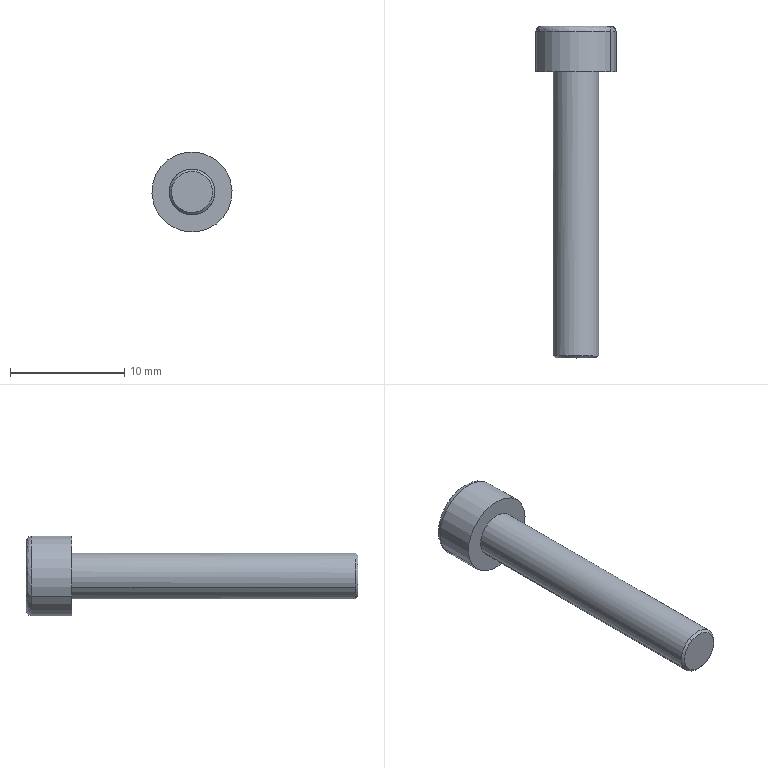Component | SolidWorks | M4X25-2 | 1 solid | 25 faces | box 7 x 29 x 7 mm | volume 449 mm3 | plane 15 | cylinder 4 | cone 4 | spline 2 | commonest cylinder face diameters 4 x2 7 x2 | material Standard Part
STEP:
#1=CARTESIAN_POINT('',(-0.3669,2.121,-0.7185));
#2=VERTEX_POINT('',#1);
#3=CARTESIAN_POINT('',(-0.6056,2.121,-0.8563));
#4=VERTEX_POINT('',#3);
#5=CARTESIAN_POINT('',(-0.4863,2.121,-0.7874));
#6=DIRECTION('',(-0.,-1.,0.));
#7=DIRECTION('',(0.866,0.,0.5));
#8=AXIS2_PLACEMENT_3D('',#5,#6,#7);
#9=CIRCLE('',#8,0.1378);
#10=EDGE_CURVE('',#2,#4,#9,.T.);
#11=ORIENTED_EDGE('',*,*,#10,.F.);
#12=CARTESIAN_POINT('',(-0.384,2.14,-0.7283));
#13=VERTEX_POINT('',#12);
#14=CARTESIAN_POINT('',(-0.384,2.121,-0.7283));
#15=DIRECTION('',(-0.5,0.,0.866));
#16=DIRECTION('',(0.866,0.,0.5));
#17=AXIS2_PLACEMENT_3D('',#14,#15,#16);
#18=CIRCLE('',#17,0.01969);
#19=EDGE_CURVE('',#2,#13,#18,.T.);
#20=ORIENTED_EDGE('',*,*,#19,.T.);
#21=CARTESIAN_POINT('',(-0.5885,2.14,-0.8465));
#22=VERTEX_POINT('',#21);
#23=CARTESIAN_POINT('',(-0.384,2.14,-0.7283));
#24=CARTESIAN_POINT('',(-0.5021,2.14,-0.5238));
#25=CARTESIAN_POINT('',(-0.7066,2.14,-0.6419));
#26=CARTESIAN_POINT('',(-0.5885,2.14,-0.8465));
#27=(BOUNDED_CURVE()B_SPLINE_CURVE(3,(#23,#24,#25,#26),.UNSPECIFIED.,.F.,.F.)B_SPLINE_CURVE_WITH_KNOTS((4,4),(0.,1.),.UNSPECIFIED.)CURVE()GEOMETRIC_REPRESENTATION_ITEM()RATIONAL_B_SPLINE_CURVE((1.,0.3333,0.3333,1.))REPRESENTATION_ITEM(''));
#28=EDGE_CURVE('',#13,#22,#27,.T.);
#29=ORIENTED_EDGE('',*,*,#28,.T.);
#30=CARTESIAN_POINT('',(-0.5885,2.121,-0.8465));
#31=DIRECTION('',(0.5,-0.,-0.866));
#32=DIRECTION('',(-0.866,0.,-0.5));
#33=AXIS2_PLACEMENT_3D('',#30,#31,#32);
#34=CIRCLE('',#33,0.01969);
#35=EDGE_CURVE('',#4,#22,#34,.T.);
#36=ORIENTED_EDGE('',*,*,#35,.F.);
#37=EDGE_LOOP('',(#11,#20,#29,#36));
#38=FACE_OUTER_BOUND('',#37,.T.);
#39=CARTESIAN_POINT('',(-0.3669,2.121,-0.7185));
#40=CARTESIAN_POINT('',(-0.5047,2.121,-0.4798));
#41=CARTESIAN_POINT('',(-0.7434,2.121,-0.6176));
#42=CARTESIAN_POINT('',(-0.6056,2.121,-0.8563));
#43=CARTESIAN_POINT('',(-0.3669,2.132,-0.7185));
#44=CARTESIAN_POINT('',(-0.5047,2.132,-0.4798));
#45=CARTESIAN_POINT('',(-0.7434,2.132,-0.6176));
#46=CARTESIAN_POINT('',(-0.6056,2.132,-0.8563));
#47=CARTESIAN_POINT('',(-0.374,2.14,-0.7226));
#48=CARTESIAN_POINT('',(-0.5036,2.14,-0.498));
#49=CARTESIAN_POINT('',(-0.7282,2.14,-0.6277));
#50=CARTESIAN_POINT('',(-0.5985,2.14,-0.8522));
#51=CARTESIAN_POINT('',(-0.384,2.14,-0.7283));
#52=CARTESIAN_POINT('',(-0.5021,2.14,-0.5238));
#53=CARTESIAN_POINT('',(-0.7066,2.14,-0.6419));
#54=CARTESIAN_POINT('',(-0.5885,2.14,-0.8465));
#55=(BOUNDED_SURFACE()B_SPLINE_SURFACE(3,3,((#39,#40,#41,#42),(#43,#44,#45,#46),(#47,#48,#49,#50),(#51,#52,#53,#54)),.UNSPECIFIED.,.F.,.F.,.T.)B_SPLINE_SURFACE_WITH_KNOTS((4,4),(4,4),(0.,1.),(0.,1.),.UNSPECIFIED.)GEOMETRIC_REPRESENTATION_ITEM()RATIONAL_B_SPLINE_SURFACE(((1.,0.3333,0.3333,1.),(0.8047,0.2682,0.2682,0.8047),(0.8047,0.2682,0.2682,0.8047),(1.,0.3333,0.3333,1.)))REPRESENTATION_ITEM('')SURFACE());
#56=ADVANCED_FACE('',(#38),#55,.T.);
#57=CARTESIAN_POINT('',(-0.4469,1.006,-0.8556));
#58=VERTEX_POINT('',#57);
#59=CARTESIAN_POINT('',(-0.5544,1.006,-0.8268));
#60=VERTEX_POINT('',#59);
#61=CARTESIAN_POINT('',(-0.4863,1.006,-0.7874));
#62=DIRECTION('',(0.,1.,-0.));
#63=DIRECTION('',(0.866,0.,0.5));
#64=AXIS2_PLACEMENT_3D('',#61,#62,#63);
#65=CIRCLE('',#64,0.07874);
#66=EDGE_CURVE('',#58,#60,#65,.T.);
#67=ORIENTED_EDGE('',*,*,#66,.T.);
#68=CARTESIAN_POINT('',(-0.5544,1.983,-0.8268));
#69=VERTEX_POINT('',#68);
#70=CARTESIAN_POINT('',(-0.5544,0.9986,-0.8268));
#71=DIRECTION('',(0.,1.,-0.));
#72=VECTOR('',#71,39.37);
#73=LINE('',#70,#72);
#74=EDGE_CURVE('',#60,#69,#73,.T.);
#75=ORIENTED_EDGE('',*,*,#74,.T.);
#76=CARTESIAN_POINT('',(-0.4181,1.983,-0.748));
#77=VERTEX_POINT('',#76);
#78=CARTESIAN_POINT('',(-0.4863,1.983,-0.7874));
#79=DIRECTION('',(-0.,-1.,0.));
#80=DIRECTION('',(0.866,0.,0.5));
#81=AXIS2_PLACEMENT_3D('',#78,#79,#80);
#82=CIRCLE('',#81,0.07874);
#83=EDGE_CURVE('',#69,#77,#82,.T.);
#84=ORIENTED_EDGE('',*,*,#83,.T.);
#85=CARTESIAN_POINT('',(-0.4181,1.006,-0.748));
#86=VERTEX_POINT('',#85);
#87=CARTESIAN_POINT('',(-0.4181,0.9986,-0.748));
#88=DIRECTION('',(0.,1.,-0.));
#89=VECTOR('',#88,39.37);
#90=LINE('',#87,#89);
#91=EDGE_CURVE('',#86,#77,#90,.T.);
#92=ORIENTED_EDGE('',*,*,#91,.F.);
#93=CARTESIAN_POINT('',(-0.4863,1.006,-0.7874));
#94=DIRECTION('',(0.,1.,-0.));
#95=DIRECTION('',(0.866,0.,0.5));
#96=AXIS2_PLACEMENT_3D('',#93,#94,#95);
#97=CIRCLE('',#96,0.07874);
#98=EDGE_CURVE('',#86,#58,#97,.T.);
#99=ORIENTED_EDGE('',*,*,#98,.T.);
#100=EDGE_LOOP('',(#67,#75,#84,#92,#99));
#101=FACE_OUTER_BOUND('',#100,.T.);
#102=CARTESIAN_POINT('',(-0.4863,0.9986,-0.7874));
#103=DIRECTION('',(0.,1.,-0.));
#104=DIRECTION('',(0.866,0.,0.5));
#105=AXIS2_PLACEMENT_3D('',#102,#103,#104);
#106=CYLINDRICAL_SURFACE('',#105,0.07874);
#107=ADVANCED_FACE('',(#101),#106,.T.);
#108=CARTESIAN_POINT('',(-0.5217,0.9986,-0.726));
#109=VERTEX_POINT('',#108);
#110=CARTESIAN_POINT('',(-0.4508,0.9986,-0.8488));
#111=VERTEX_POINT('',#110);
#112=CARTESIAN_POINT('',(-0.4863,0.9986,-0.7874));
#113=DIRECTION('',(-0.,1.,0.));
#114=DIRECTION('',(-0.5,0.,0.866));
#115=AXIS2_PLACEMENT_3D('',#112,#113,#114);
#116=CIRCLE('',#115,0.07087);
#117=EDGE_CURVE('',#109,#111,#116,.T.);
#118=ORIENTED_EDGE('',*,*,#117,.T.);
#119=CARTESIAN_POINT('',(-0.4469,1.006,-0.8556));
#120=DIRECTION('',(0.3536,0.7071,-0.6124));
#121=VECTOR('',#120,39.37);
#122=LINE('',#119,#121);
#123=EDGE_CURVE('',#111,#58,#122,.T.);
#124=ORIENTED_EDGE('',*,*,#123,.T.);
#125=ORIENTED_EDGE('',*,*,#98,.F.);
#126=CARTESIAN_POINT('',(-0.5256,1.006,-0.7192));
#127=VERTEX_POINT('',#126);
#128=CARTESIAN_POINT('',(-0.4863,1.006,-0.7874));
#129=DIRECTION('',(0.,1.,-0.));
#130=DIRECTION('',(0.866,0.,0.5));
#131=AXIS2_PLACEMENT_3D('',#128,#129,#130);
#132=CIRCLE('',#131,0.07874);
#133=EDGE_CURVE('',#127,#86,#132,.T.);
#134=ORIENTED_EDGE('',*,*,#133,.F.);
#135=CARTESIAN_POINT('',(-0.5256,1.006,-0.7192));
#136=DIRECTION('',(-0.3536,0.7071,0.6124));
#137=VECTOR('',#136,39.37);
#138=LINE('',#135,#137);
#139=EDGE_CURVE('',#109,#127,#138,.T.);
#140=ORIENTED_EDGE('',*,*,#139,.F.);
#141=EDGE_LOOP('',(#118,#124,#125,#134,#140));
#142=FACE_OUTER_BOUND('',#141,.T.);
#143=CARTESIAN_POINT('',(-0.4863,1.006,-0.7874));
#144=DIRECTION('',(-0.,1.,0.));
#145=DIRECTION('',(-0.5,0.,0.866));
#146=AXIS2_PLACEMENT_3D('',#143,#144,#145);
#147=CONICAL_SURFACE('',#146,0.07874,0.7854);
#148=ADVANCED_FACE('',(#142),#147,.T.);
#149=CARTESIAN_POINT('',(-0.6056,1.983,-0.8563));
#150=VERTEX_POINT('',#149);
#151=CARTESIAN_POINT('',(-0.3669,1.983,-0.7185));
#152=VERTEX_POINT('',#151);
#153=CARTESIAN_POINT('',(-0.4863,1.983,-0.7874));
#154=DIRECTION('',(-0.,-1.,0.));
#155=DIRECTION('',(0.866,0.,0.5));
#156=AXIS2_PLACEMENT_3D('',#153,#154,#155);
#157=CIRCLE('',#156,0.1378);
#158=EDGE_CURVE('',#150,#152,#157,.T.);
#159=ORIENTED_EDGE('',*,*,#158,.F.);
#160=CARTESIAN_POINT('',(-0.6056,1.983,-0.8563));
#161=DIRECTION('',(0.,1.,-0.));
#162=VECTOR('',#161,39.37);
#163=LINE('',#160,#162);
#164=EDGE_CURVE('',#150,#4,#163,.T.);
#165=ORIENTED_EDGE('',*,*,#164,.T.);
#166=CARTESIAN_POINT('',(-0.4863,2.121,-0.7874));
#167=DIRECTION('',(-0.,-1.,0.));
#168=DIRECTION('',(0.866,0.,0.5));
#169=AXIS2_PLACEMENT_3D('',#166,#167,#168);
#170=CIRCLE('',#169,0.1378);
#171=EDGE_CURVE('',#4,#2,#170,.T.);
#172=ORIENTED_EDGE('',*,*,#171,.T.);
#173=CARTESIAN_POINT('',(-0.3669,1.983,-0.7185));
#174=DIRECTION('',(0.,1.,-0.));
#175=VECTOR('',#174,39.37);
#176=LINE('',#173,#175);
#177=EDGE_CURVE('',#152,#2,#176,.T.);
#178=ORIENTED_EDGE('',*,*,#177,.F.);
#179=EDGE_LOOP('',(#159,#165,#172,#178));
#180=FACE_OUTER_BOUND('',#179,.T.);
#181=CARTESIAN_POINT('',(-0.4863,1.983,-0.7874));
#182=DIRECTION('',(0.,1.,-0.));
#183=DIRECTION('',(0.866,0.,0.5));
#184=AXIS2_PLACEMENT_3D('',#181,#182,#183);
#185=CYLINDRICAL_SURFACE('',#184,0.1378);
#186=ADVANCED_FACE('',(#180),#185,.T.);
#187=CARTESIAN_POINT('',(-0.4863,2.027,-0.7874));
#188=VERTEX_POINT('',#187);
#189=CARTESIAN_POINT('',(-0.4351,2.062,-0.7579));
#190=VERTEX_POINT('',#189);
#191=CARTESIAN_POINT('',(-0.4351,2.062,-0.7579));
#192=DIRECTION('',(0.75,0.5,0.433));
#193=VECTOR('',#192,39.37);
#194=LINE('',#191,#193);
#195=EDGE_CURVE('',#188,#190,#194,.T.);
#196=ORIENTED_EDGE('',*,*,#195,.F.);
#197=CARTESIAN_POINT('',(-0.5374,2.062,-0.8169));
#198=VERTEX_POINT('',#197);
#199=CARTESIAN_POINT('',(-0.5374,2.062,-0.8169));
#200=DIRECTION('',(-0.75,0.5,-0.433));
#201=VECTOR('',#200,39.37);
#202=LINE('',#199,#201);
#203=EDGE_CURVE('',#188,#198,#202,.T.);
#204=ORIENTED_EDGE('',*,*,#203,.T.);
#205=CARTESIAN_POINT('',(-0.5453,2.062,-0.7874));
#206=VERTEX_POINT('',#205);
#207=CARTESIAN_POINT('',(-0.4863,2.062,-0.7874));
#208=DIRECTION('',(-0.,-1.,0.));
#209=DIRECTION('',(0.866,0.,0.5));
#210=AXIS2_PLACEMENT_3D('',#207,#208,#209);
#211=CIRCLE('',#210,0.05906);
#212=EDGE_CURVE('',#206,#198,#211,.T.);
#213=ORIENTED_EDGE('',*,*,#212,.F.);
#214=CARTESIAN_POINT('',(-0.5158,2.062,-0.7363));
#215=VERTEX_POINT('',#214);
#216=CARTESIAN_POINT('',(-0.4863,2.062,-0.7874));
#217=DIRECTION('',(0.,1.,-0.));
#218=DIRECTION('',(0.866,0.,0.5));
#219=AXIS2_PLACEMENT_3D('',#216,#217,#218);
#220=CIRCLE('',#219,0.05906);
#221=EDGE_CURVE('',#206,#215,#220,.T.);
#222=ORIENTED_EDGE('',*,*,#221,.T.);
#223=CARTESIAN_POINT('',(-0.4567,2.062,-0.7363));
#224=VERTEX_POINT('',#223);
#225=CARTESIAN_POINT('',(-0.4863,2.062,-0.7874));
#226=DIRECTION('',(-0.,-1.,0.));
#227=DIRECTION('',(0.866,0.,0.5));
#228=AXIS2_PLACEMENT_3D('',#225,#226,#227);
#229=CIRCLE('',#228,0.05906);
#230=EDGE_CURVE('',#224,#215,#229,.T.);
#231=ORIENTED_EDGE('',*,*,#230,.F.);
#232=CARTESIAN_POINT('',(-0.4863,2.062,-0.7874));
#233=DIRECTION('',(-0.,-1.,0.));
#234=DIRECTION('',(0.866,0.,0.5));
#235=AXIS2_PLACEMENT_3D('',#232,#233,#234);
#236=CIRCLE('',#235,0.05906);
#237=EDGE_CURVE('',#190,#224,#236,.T.);
#238=ORIENTED_EDGE('',*,*,#237,.F.);
#239=EDGE_LOOP('',(#196,#204,#213,#222,#231,#238));
#240=FACE_OUTER_BOUND('',#239,.T.);
#241=CARTESIAN_POINT('',(-0.4863,2.062,-0.7874));
#242=DIRECTION('',(0.,1.,-0.));
#243=DIRECTION('',(0.866,0.,0.5));
#244=AXIS2_PLACEMENT_3D('',#241,#242,#243);
#245=CONICAL_SURFACE('',#244,0.05906,1.047);
#246=ADVANCED_FACE('',(#240),#245,.F.);
#247=ORIENTED_EDGE('',*,*,#74,.F.);
#248=CARTESIAN_POINT('',(-0.4863,1.006,-0.7874));
#249=DIRECTION('',(0.,1.,-0.));
#250=DIRECTION('',(0.866,0.,0.5));
#251=AXIS2_PLACEMENT_3D('',#248,#249,#250);
#252=CIRCLE('',#251,0.07874);
#253=EDGE_CURVE('',#60,#127,#252,.T.);
#254=ORIENTED_EDGE('',*,*,#253,.T.);
#255=ORIENTED_EDGE('',*,*,#133,.T.);
#256=ORIENTED_EDGE('',*,*,#91,.T.);
#257=CARTESIAN_POINT('',(-0.4863,1.983,-0.7874));
#258=DIRECTION('',(-0.,-1.,0.));
#259=DIRECTION('',(0.866,0.,0.5));
#260=AXIS2_PLACEMENT_3D('',#257,#258,#259);
#261=CIRCLE('',#260,0.07874);
#262=EDGE_CURVE('',#77,#69,#261,.T.);
#263=ORIENTED_EDGE('',*,*,#262,.T.);
#264=EDGE_LOOP('',(#247,#254,#255,#256,#263));
#265=FACE_OUTER_BOUND('',#264,.T.);
#266=CARTESIAN_POINT('',(-0.4863,0.9986,-0.7874));
#267=DIRECTION('',(0.,1.,-0.));
#268=DIRECTION('',(0.866,0.,0.5));
#269=AXIS2_PLACEMENT_3D('',#266,#267,#268);
#270=CYLINDRICAL_SURFACE('',#269,0.07874);
#271=ADVANCED_FACE('',(#265),#270,.T.);
#272=ORIENTED_EDGE('',*,*,#262,.F.);
#273=ORIENTED_EDGE('',*,*,#83,.F.);
#274=EDGE_LOOP('',(#272,#273));
#275=FACE_BOUND('',#274,.T.);
#276=CARTESIAN_POINT('',(-0.4863,1.983,-0.7874));
#277=DIRECTION('',(-0.,-1.,0.));
#278=DIRECTION('',(0.866,0.,0.5));
#279=AXIS2_PLACEMENT_3D('',#276,#277,#278);
#280=CIRCLE('',#279,0.1378);
#281=EDGE_CURVE('',#152,#150,#280,.T.);
#282=ORIENTED_EDGE('',*,*,#281,.T.);
#283=ORIENTED_EDGE('',*,*,#158,.T.);
#284=EDGE_LOOP('',(#282,#283));
#285=FACE_OUTER_BOUND('',#284,.T.);
#286=CARTESIAN_POINT('',(-0.4863,1.983,-0.7874));
#287=DIRECTION('',(-0.,-1.,0.));
#288=DIRECTION('',(-0.866,0.,-0.5));
#289=AXIS2_PLACEMENT_3D('',#286,#287,#288);
#290=PLANE('',#289);
#291=ADVANCED_FACE('',(#275,#285),#290,.T.);
#292=ORIENTED_EDGE('',*,*,#123,.F.);
#293=CARTESIAN_POINT('',(-0.4863,0.9986,-0.7874));
#294=DIRECTION('',(-0.,1.,0.));
#295=DIRECTION('',(-0.5,0.,0.866));
#296=AXIS2_PLACEMENT_3D('',#293,#294,#295);
#297=CIRCLE('',#296,0.07087);
#298=EDGE_CURVE('',#111,#109,#297,.T.);
#299=ORIENTED_EDGE('',*,*,#298,.T.);
#300=ORIENTED_EDGE('',*,*,#139,.T.);
#301=ORIENTED_EDGE('',*,*,#253,.F.);
#302=ORIENTED_EDGE('',*,*,#66,.F.);
#303=EDGE_LOOP('',(#292,#299,#300,#301,#302));
#304=FACE_OUTER_BOUND('',#303,.T.);
#305=CARTESIAN_POINT('',(-0.4863,1.006,-0.7874));
#306=DIRECTION('',(-0.,1.,0.));
#307=DIRECTION('',(-0.5,0.,0.866));
#308=AXIS2_PLACEMENT_3D('',#305,#306,#307);
#309=CONICAL_SURFACE('',#308,0.07874,0.7854);
#310=ADVANCED_FACE('',(#304),#309,.T.);
#311=ORIENTED_EDGE('',*,*,#164,.F.);
#312=ORIENTED_EDGE('',*,*,#281,.F.);
#313=ORIENTED_EDGE('',*,*,#177,.T.);
#314=ORIENTED_EDGE('',*,*,#10,.T.);
#315=EDGE_LOOP('',(#311,#312,#313,#314));
#316=FACE_OUTER_BOUND('',#315,.T.);
#317=CARTESIAN_POINT('',(-0.4863,1.983,-0.7874));
#318=DIRECTION('',(0.,1.,-0.));
#319=DIRECTION('',(0.866,0.,0.5));
#320=AXIS2_PLACEMENT_3D('',#317,#318,#319);
#321=CYLINDRICAL_SURFACE('',#320,0.1378);
#322=ADVANCED_FACE('',(#316),#321,.T.);
#323=ORIENTED_EDGE('',*,*,#117,.F.);
#324=ORIENTED_EDGE('',*,*,#298,.F.);
#325=EDGE_LOOP('',(#323,#324));
#326=FACE_OUTER_BOUND('',#325,.T.);
#327=CARTESIAN_POINT('',(-0.4863,0.9986,-0.7874));
#328=DIRECTION('',(-0.,-1.,0.));
#329=DIRECTION('',(-0.866,0.,-0.5));
#330=AXIS2_PLACEMENT_3D('',#327,#328,#329);
#331=PLANE('',#330);
#332=ADVANCED_FACE('',(#326),#331,.T.);
#333=ORIENTED_EDGE('',*,*,#19,.F.);
#334=ORIENTED_EDGE('',*,*,#171,.F.);
#335=ORIENTED_EDGE('',*,*,#35,.T.);
#336=CARTESIAN_POINT('',(-0.5885,2.14,-0.8465));
#337=CARTESIAN_POINT('',(-0.4704,2.14,-1.051));
#338=CARTESIAN_POINT('',(-0.2659,2.14,-0.9329));
#339=CARTESIAN_POINT('',(-0.384,2.14,-0.7283));
#340=(BOUNDED_CURVE()B_SPLINE_CURVE(3,(#336,#337,#338,#339),.UNSPECIFIED.,.F.,.F.)B_SPLINE_CURVE_WITH_KNOTS((4,4),(0.,1.),.UNSPECIFIED.)CURVE()GEOMETRIC_REPRESENTATION_ITEM()RATIONAL_B_SPLINE_CURVE((1.,0.3333,0.3333,1.))REPRESENTATION_ITEM(''));
#341=EDGE_CURVE('',#22,#13,#340,.T.);
#342=ORIENTED_EDGE('',*,*,#341,.T.);
#343=EDGE_LOOP('',(#333,#334,#335,#342));
#344=FACE_OUTER_BOUND('',#343,.T.);
#345=CARTESIAN_POINT('',(-0.6056,2.121,-0.8563));
#346=CARTESIAN_POINT('',(-0.4678,2.121,-1.095));
#347=CARTESIAN_POINT('',(-0.2291,2.121,-0.9572));
#348=CARTESIAN_POINT('',(-0.3669,2.121,-0.7185));
#349=CARTESIAN_POINT('',(-0.6056,2.132,-0.8563));
#350=CARTESIAN_POINT('',(-0.4678,2.132,-1.095));
#351=CARTESIAN_POINT('',(-0.2291,2.132,-0.9572));
#352=CARTESIAN_POINT('',(-0.3669,2.132,-0.7185));
#353=CARTESIAN_POINT('',(-0.5985,2.14,-0.8522));
#354=CARTESIAN_POINT('',(-0.4689,2.14,-1.077));
#355=CARTESIAN_POINT('',(-0.2443,2.14,-0.9471));
#356=CARTESIAN_POINT('',(-0.374,2.14,-0.7226));
#357=CARTESIAN_POINT('',(-0.5885,2.14,-0.8465));
#358=CARTESIAN_POINT('',(-0.4704,2.14,-1.051));
#359=CARTESIAN_POINT('',(-0.2659,2.14,-0.9329));
#360=CARTESIAN_POINT('',(-0.384,2.14,-0.7283));
#361=(BOUNDED_SURFACE()B_SPLINE_SURFACE(3,3,((#345,#346,#347,#348),(#349,#350,#351,#352),(#353,#354,#355,#356),(#357,#358,#359,#360)),.UNSPECIFIED.,.F.,.F.,.T.)B_SPLINE_SURFACE_WITH_KNOTS((4,4),(4,4),(0.,1.),(0.,1.),.UNSPECIFIED.)GEOMETRIC_REPRESENTATION_ITEM()RATIONAL_B_SPLINE_SURFACE(((1.,0.3333,0.3333,1.),(0.8047,0.2682,0.2682,0.8047),(0.8047,0.2682,0.2682,0.8047),(1.,0.3333,0.3333,1.)))REPRESENTATION_ITEM('')SURFACE());
#362=ADVANCED_FACE('',(#344),#361,.T.);
#363=CARTESIAN_POINT('',(-0.4863,2.14,-0.8556));
#364=VERTEX_POINT('',#363);
#365=CARTESIAN_POINT('',(-0.5453,2.14,-0.8215));
#366=VERTEX_POINT('',#365);
#367=CARTESIAN_POINT('',(-0.5453,2.14,-0.8215));
#368=DIRECTION('',(-0.866,0.,0.5));
#369=VECTOR('',#368,39.37);
#370=LINE('',#367,#369);
#371=EDGE_CURVE('',#364,#366,#370,.T.);
#372=ORIENTED_EDGE('',*,*,#371,.F.);
#373=CARTESIAN_POINT('',(-0.4272,2.14,-0.8215));
#374=VERTEX_POINT('',#373);
#375=CARTESIAN_POINT('',(-0.4863,2.14,-0.8556));
#376=DIRECTION('',(-0.866,0.,-0.5));
#377=VECTOR('',#376,39.37);
#378=LINE('',#375,#377);
#379=EDGE_CURVE('',#374,#364,#378,.T.);
#380=ORIENTED_EDGE('',*,*,#379,.F.);
#381=CARTESIAN_POINT('',(-0.4272,2.14,-0.7533));
#382=VERTEX_POINT('',#381);
#383=CARTESIAN_POINT('',(-0.4272,2.14,-0.8215));
#384=DIRECTION('',(-0.,-0.,-1.));
#385=VECTOR('',#384,39.37);
#386=LINE('',#383,#385);
#387=EDGE_CURVE('',#382,#374,#386,.T.);
#388=ORIENTED_EDGE('',*,*,#387,.F.);
#389=CARTESIAN_POINT('',(-0.4863,2.14,-0.7192));
#390=VERTEX_POINT('',#389);
#391=CARTESIAN_POINT('',(-0.4272,2.14,-0.7533));
#392=DIRECTION('',(0.866,-0.,-0.5));
#393=VECTOR('',#392,39.37);
#394=LINE('',#391,#393);
#395=EDGE_CURVE('',#390,#382,#394,.T.);
#396=ORIENTED_EDGE('',*,*,#395,.F.);
#397=CARTESIAN_POINT('',(-0.5453,2.14,-0.7533));
#398=VERTEX_POINT('',#397);
#399=CARTESIAN_POINT('',(-0.4863,2.14,-0.7192));
#400=DIRECTION('',(0.866,-0.,0.5));
#401=VECTOR('',#400,39.37);
#402=LINE('',#399,#401);
#403=EDGE_CURVE('',#398,#390,#402,.T.);
#404=ORIENTED_EDGE('',*,*,#403,.F.);
#405=CARTESIAN_POINT('',(-0.5453,2.14,-0.8215));
#406=DIRECTION('',(0.,0.,1.));
#407=VECTOR('',#406,39.37);
#408=LINE('',#405,#407);
#409=EDGE_CURVE('',#366,#398,#408,.T.);
#410=ORIENTED_EDGE('',*,*,#409,.F.);
#411=EDGE_LOOP('',(#372,#380,#388,#396,#404,#410));
#412=FACE_BOUND('',#411,.T.);
#413=ORIENTED_EDGE('',*,*,#341,.F.);
#414=ORIENTED_EDGE('',*,*,#28,.F.);
#415=EDGE_LOOP('',(#413,#414));
#416=FACE_OUTER_BOUND('',#415,.T.);
#417=CARTESIAN_POINT('',(-0.4863,2.14,-0.7874));
#418=DIRECTION('',(-0.,-1.,0.));
#419=DIRECTION('',(-0.866,0.,-0.5));
#420=AXIS2_PLACEMENT_3D('',#417,#418,#419);
#421=PLANE('',#420);
#422=ADVANCED_FACE('',(#412,#416),#421,.F.);
#423=CARTESIAN_POINT('',(-0.5453,2.062,-0.8215));
#424=VERTEX_POINT('',#423);
#425=CARTESIAN_POINT('',(-0.5453,2.062,-0.7533));
#426=DIRECTION('',(0.,-0.,-1.));
#427=VECTOR('',#426,39.37);
#428=LINE('',#425,#427);
#429=EDGE_CURVE('',#206,#424,#428,.T.);
#430=ORIENTED_EDGE('',*,*,#429,.T.);
#431=CARTESIAN_POINT('',(-0.5453,2.062,-0.8215));
#432=DIRECTION('',(0.,1.,-0.));
#433=VECTOR('',#432,39.37);
#434=LINE('',#431,#433);
#435=EDGE_CURVE('',#424,#366,#434,.T.);
#436=ORIENTED_EDGE('',*,*,#435,.T.);
#437=ORIENTED_EDGE('',*,*,#409,.T.);
#438=CARTESIAN_POINT('',(-0.5453,2.062,-0.7533));
#439=VERTEX_POINT('',#438);
#440=CARTESIAN_POINT('',(-0.5453,2.062,-0.7533));
#441=DIRECTION('',(-0.,-1.,0.));
#442=VECTOR('',#441,39.37);
#443=LINE('',#440,#442);
#444=EDGE_CURVE('',#398,#439,#443,.T.);
#445=ORIENTED_EDGE('',*,*,#444,.T.);
#446=CARTESIAN_POINT('',(-0.5453,2.062,-0.7533));
#447=DIRECTION('',(0.,-0.,-1.));
#448=VECTOR('',#447,39.37);
#449=LINE('',#446,#448);
#450=EDGE_CURVE('',#439,#206,#449,.T.);
#451=ORIENTED_EDGE('',*,*,#450,.T.);
#452=EDGE_LOOP('',(#430,#436,#437,#445,#451));
#453=FACE_OUTER_BOUND('',#452,.T.);
#454=CARTESIAN_POINT('',(-0.5453,2.062,-0.7533));
#455=DIRECTION('',(1.,-0.,0.));
#456=DIRECTION('',(0.,0.,1.));
#457=AXIS2_PLACEMENT_3D('',#454,#455,#456);
#458=PLANE('',#457);
#459=ADVANCED_FACE('',(#453),#458,.T.);
#460=CARTESIAN_POINT('',(-0.5158,2.062,-0.8385));
#461=VERTEX_POINT('',#460);
#462=CARTESIAN_POINT('',(-0.4863,2.062,-0.8556));
#463=VERTEX_POINT('',#462);
#464=CARTESIAN_POINT('',(-0.5453,2.062,-0.8215));
#465=DIRECTION('',(0.866,-0.,-0.5));
#466=VECTOR('',#465,39.37);
#467=LINE('',#464,#466);
#468=EDGE_CURVE('',#461,#463,#467,.T.);
#469=ORIENTED_EDGE('',*,*,#468,.T.);
#470=CARTESIAN_POINT('',(-0.4863,2.062,-0.8556));
#471=DIRECTION('',(0.,1.,-0.));
#472=VECTOR('',#471,39.37);
#473=LINE('',#470,#472);
#474=EDGE_CURVE('',#463,#364,#473,.T.);
#475=ORIENTED_EDGE('',*,*,#474,.T.);
#476=ORIENTED_EDGE('',*,*,#371,.T.);
#477=ORIENTED_EDGE('',*,*,#435,.F.);
#478=CARTESIAN_POINT('',(-0.5453,2.062,-0.8215));
#479=DIRECTION('',(0.866,-0.,-0.5));
#480=VECTOR('',#479,39.37);
#481=LINE('',#478,#480);
#482=EDGE_CURVE('',#424,#461,#481,.T.);
#483=ORIENTED_EDGE('',*,*,#482,.T.);
#484=EDGE_LOOP('',(#469,#475,#476,#477,#483));
#485=FACE_OUTER_BOUND('',#484,.T.);
#486=CARTESIAN_POINT('',(-0.5453,2.062,-0.8215));
#487=DIRECTION('',(0.5,0.,0.866));
#488=DIRECTION('',(-0.866,0.,0.5));
#489=AXIS2_PLACEMENT_3D('',#486,#487,#488);
#490=PLANE('',#489);
#491=ADVANCED_FACE('',(#485),#490,.T.);
#492=ORIENTED_EDGE('',*,*,#482,.F.);
#493=ORIENTED_EDGE('',*,*,#429,.F.);
#494=ORIENTED_EDGE('',*,*,#212,.T.);
#495=CARTESIAN_POINT('',(-0.4863,2.062,-0.7874));
#496=DIRECTION('',(-0.,-1.,0.));
#497=DIRECTION('',(0.866,0.,0.5));
#498=AXIS2_PLACEMENT_3D('',#495,#496,#497);
#499=CIRCLE('',#498,0.05906);
#500=EDGE_CURVE('',#198,#461,#499,.T.);
#501=ORIENTED_EDGE('',*,*,#500,.T.);
#502=EDGE_LOOP('',(#492,#493,#494,#501));
#503=FACE_OUTER_BOUND('',#502,.T.);
#504=CARTESIAN_POINT('',(-0.5453,2.062,-0.8897));
#505=DIRECTION('',(-0.,-1.,0.));
#506=DIRECTION('',(-0.866,0.,-0.5));
#507=AXIS2_PLACEMENT_3D('',#504,#505,#506);
#508=PLANE('',#507);
#509=ADVANCED_FACE('',(#503),#508,.F.);
#510=ORIENTED_EDGE('',*,*,#450,.F.);
#511=CARTESIAN_POINT('',(-0.6044,2.062,-0.7874));
#512=DIRECTION('',(-0.866,0.,-0.5));
#513=VECTOR('',#512,39.37);
#514=LINE('',#511,#513);
#515=EDGE_CURVE('',#215,#439,#514,.T.);
#516=ORIENTED_EDGE('',*,*,#515,.F.);
#517=ORIENTED_EDGE('',*,*,#221,.F.);
#518=EDGE_LOOP('',(#510,#516,#517));
#519=FACE_OUTER_BOUND('',#518,.T.);
#520=CARTESIAN_POINT('',(-0.5453,2.062,-0.8897));
#521=DIRECTION('',(-0.,-1.,0.));
#522=DIRECTION('',(-0.866,0.,-0.5));
#523=AXIS2_PLACEMENT_3D('',#520,#521,#522);
#524=PLANE('',#523);
#525=ADVANCED_FACE('',(#519),#524,.F.);
#526=ORIENTED_EDGE('',*,*,#515,.T.);
#527=ORIENTED_EDGE('',*,*,#444,.F.);
#528=ORIENTED_EDGE('',*,*,#403,.T.);
#529=CARTESIAN_POINT('',(-0.4863,2.062,-0.7192));
#530=VERTEX_POINT('',#529);
#531=CARTESIAN_POINT('',(-0.4863,2.062,-0.7192));
#532=DIRECTION('',(-0.,-1.,0.));
#533=VECTOR('',#532,39.37);
#534=LINE('',#531,#533);
#535=EDGE_CURVE('',#390,#530,#534,.T.);
#536=ORIENTED_EDGE('',*,*,#535,.T.);
#537=CARTESIAN_POINT('',(-0.4863,2.062,-0.7192));
#538=DIRECTION('',(-0.866,0.,-0.5));
#539=VECTOR('',#538,39.37);
#540=LINE('',#537,#539);
#541=EDGE_CURVE('',#530,#215,#540,.T.);
#542=ORIENTED_EDGE('',*,*,#541,.T.);
#543=EDGE_LOOP('',(#526,#527,#528,#536,#542));
#544=FACE_OUTER_BOUND('',#543,.T.);
#545=CARTESIAN_POINT('',(-0.4863,2.062,-0.7192));
#546=DIRECTION('',(0.5,-0.,-0.866));
#547=DIRECTION('',(0.866,-0.,0.5));
#548=AXIS2_PLACEMENT_3D('',#545,#546,#547);
#549=PLANE('',#548);
#550=ADVANCED_FACE('',(#544),#549,.T.);
#551=CARTESIAN_POINT('',(-0.4567,2.062,-0.8385));
#552=VERTEX_POINT('',#551);
#553=CARTESIAN_POINT('',(-0.4272,2.062,-0.8215));
#554=VERTEX_POINT('',#553);
#555=CARTESIAN_POINT('',(-0.4863,2.062,-0.8556));
#556=DIRECTION('',(0.866,-0.,0.5));
#557=VECTOR('',#556,39.37);
#558=LINE('',#555,#557);
#559=EDGE_CURVE('',#552,#554,#558,.T.);
#560=ORIENTED_EDGE('',*,*,#559,.T.);
#561=CARTESIAN_POINT('',(-0.4272,2.062,-0.8215));
#562=DIRECTION('',(0.,1.,-0.));
#563=VECTOR('',#562,39.37);
#564=LINE('',#561,#563);
#565=EDGE_CURVE('',#554,#374,#564,.T.);
#566=ORIENTED_EDGE('',*,*,#565,.T.);
#567=ORIENTED_EDGE('',*,*,#379,.T.);
#568=ORIENTED_EDGE('',*,*,#474,.F.);
#569=CARTESIAN_POINT('',(-0.4863,2.062,-0.8556));
#570=DIRECTION('',(0.866,-0.,0.5));
#571=VECTOR('',#570,39.37);
#572=LINE('',#569,#571);
#573=EDGE_CURVE('',#463,#552,#572,.T.);
#574=ORIENTED_EDGE('',*,*,#573,.T.);
#575=EDGE_LOOP('',(#560,#566,#567,#568,#574));
#576=FACE_OUTER_BOUND('',#575,.T.);
#577=CARTESIAN_POINT('',(-0.4863,2.062,-0.8556));
#578=DIRECTION('',(-0.5,0.,0.866));
#579=DIRECTION('',(-0.866,0.,-0.5));
#580=AXIS2_PLACEMENT_3D('',#577,#578,#579);
#581=PLANE('',#580);
#582=ADVANCED_FACE('',(#576),#581,.T.);
#583=ORIENTED_EDGE('',*,*,#573,.F.);
#584=ORIENTED_EDGE('',*,*,#468,.F.);
#585=CARTESIAN_POINT('',(-0.4863,2.062,-0.7874));
#586=DIRECTION('',(0.,1.,-0.));
#587=DIRECTION('',(0.866,0.,0.5));
#588=AXIS2_PLACEMENT_3D('',#585,#586,#587);
#589=CIRCLE('',#588,0.05906);
#590=EDGE_CURVE('',#552,#461,#589,.T.);
#591=ORIENTED_EDGE('',*,*,#590,.F.);
#592=EDGE_LOOP('',(#583,#584,#591));
#593=FACE_OUTER_BOUND('',#592,.T.);
#594=CARTESIAN_POINT('',(-0.5453,2.062,-0.8897));
#595=DIRECTION('',(-0.,-1.,0.));
#596=DIRECTION('',(-0.866,0.,-0.5));
#597=AXIS2_PLACEMENT_3D('',#594,#595,#596);
#598=PLANE('',#597);
#599=ADVANCED_FACE('',(#593),#598,.F.);
#600=ORIENTED_EDGE('',*,*,#203,.F.);
#601=ORIENTED_EDGE('',*,*,#195,.T.);
#602=CARTESIAN_POINT('',(-0.4272,2.062,-0.7874));
#603=VERTEX_POINT('',#602);
#604=CARTESIAN_POINT('',(-0.4863,2.062,-0.7874));
#605=DIRECTION('',(-0.,-1.,0.));
#606=DIRECTION('',(0.866,0.,0.5));
#607=AXIS2_PLACEMENT_3D('',#604,#605,#606);
#608=CIRCLE('',#607,0.05906);
#609=EDGE_CURVE('',#603,#190,#608,.T.);
#610=ORIENTED_EDGE('',*,*,#609,.F.);
#611=CARTESIAN_POINT('',(-0.4863,2.062,-0.7874));
#612=DIRECTION('',(0.,1.,-0.));
#613=DIRECTION('',(0.866,0.,0.5));
#614=AXIS2_PLACEMENT_3D('',#611,#612,#613);
#615=CIRCLE('',#614,0.05906);
#616=EDGE_CURVE('',#603,#552,#615,.T.);
#617=ORIENTED_EDGE('',*,*,#616,.T.);
#618=ORIENTED_EDGE('',*,*,#590,.T.);
#619=ORIENTED_EDGE('',*,*,#500,.F.);
#620=EDGE_LOOP('',(#600,#601,#610,#617,#618,#619));
#621=FACE_OUTER_BOUND('',#620,.T.);
#622=CARTESIAN_POINT('',(-0.4863,2.062,-0.7874));
#623=DIRECTION('',(0.,1.,-0.));
#624=DIRECTION('',(0.866,0.,0.5));
#625=AXIS2_PLACEMENT_3D('',#622,#623,#624);
#626=CONICAL_SURFACE('',#625,0.05906,1.047);
#627=ADVANCED_FACE('',(#621),#626,.F.);
#628=ORIENTED_EDGE('',*,*,#541,.F.);
#629=CARTESIAN_POINT('',(-0.4567,2.062,-0.7363));
#630=DIRECTION('',(-0.866,0.,0.5));
#631=VECTOR('',#630,39.37);
#632=LINE('',#629,#631);
#633=EDGE_CURVE('',#224,#530,#632,.T.);
#634=ORIENTED_EDGE('',*,*,#633,.F.);
#635=ORIENTED_EDGE('',*,*,#230,.T.);
#636=EDGE_LOOP('',(#628,#634,#635));
#637=FACE_OUTER_BOUND('',#636,.T.);
#638=CARTESIAN_POINT('',(-0.5453,2.062,-0.8897));
#639=DIRECTION('',(-0.,-1.,0.));
#640=DIRECTION('',(-0.866,0.,-0.5));
#641=AXIS2_PLACEMENT_3D('',#638,#639,#640);
#642=PLANE('',#641);
#643=ADVANCED_FACE('',(#637),#642,.F.);
#644=ORIENTED_EDGE('',*,*,#633,.T.);
#645=ORIENTED_EDGE('',*,*,#535,.F.);
#646=ORIENTED_EDGE('',*,*,#395,.T.);
#647=CARTESIAN_POINT('',(-0.4272,2.062,-0.7533));
#648=VERTEX_POINT('',#647);
#649=CARTESIAN_POINT('',(-0.4272,2.062,-0.7533));
#650=DIRECTION('',(-0.,-1.,0.));
#651=VECTOR('',#650,39.37);
#652=LINE('',#649,#651);
#653=EDGE_CURVE('',#382,#648,#652,.T.);
#654=ORIENTED_EDGE('',*,*,#653,.T.);
#655=CARTESIAN_POINT('',(-0.4272,2.062,-0.7533));
#656=DIRECTION('',(-0.866,0.,0.5));
#657=VECTOR('',#656,39.37);
#658=LINE('',#655,#657);
#659=EDGE_CURVE('',#648,#224,#658,.T.);
#660=ORIENTED_EDGE('',*,*,#659,.T.);
#661=EDGE_LOOP('',(#644,#645,#646,#654,#660));
#662=FACE_OUTER_BOUND('',#661,.T.);
#663=CARTESIAN_POINT('',(-0.4272,2.062,-0.7533));
#664=DIRECTION('',(-0.5,-0.,-0.866));
#665=DIRECTION('',(0.866,-0.,-0.5));
#666=AXIS2_PLACEMENT_3D('',#663,#664,#665);
#667=PLANE('',#666);
#668=ADVANCED_FACE('',(#662),#667,.T.);
#669=CARTESIAN_POINT('',(-0.4272,2.062,-0.8215));
#670=DIRECTION('',(0.,0.,1.));
#671=VECTOR('',#670,39.37);
#672=LINE('',#669,#671);
#673=EDGE_CURVE('',#603,#648,#672,.T.);
#674=ORIENTED_EDGE('',*,*,#673,.T.);
#675=ORIENTED_EDGE('',*,*,#653,.F.);
#676=ORIENTED_EDGE('',*,*,#387,.T.);
#677=ORIENTED_EDGE('',*,*,#565,.F.);
#678=CARTESIAN_POINT('',(-0.4272,2.062,-0.8215));
#679=DIRECTION('',(0.,0.,1.));
#680=VECTOR('',#679,39.37);
#681=LINE('',#678,#680);
#682=EDGE_CURVE('',#554,#603,#681,.T.);
#683=ORIENTED_EDGE('',*,*,#682,.T.);
#684=EDGE_LOOP('',(#674,#675,#676,#677,#683));
#685=FACE_OUTER_BOUND('',#684,.T.);
#686=CARTESIAN_POINT('',(-0.4272,2.062,-0.8215));
#687=DIRECTION('',(-1.,0.,0.));
#688=DIRECTION('',(-0.,-0.,-1.));
#689=AXIS2_PLACEMENT_3D('',#686,#687,#688);
#690=PLANE('',#689);
#691=ADVANCED_FACE('',(#685),#690,.T.);
#692=ORIENTED_EDGE('',*,*,#682,.F.);
#693=ORIENTED_EDGE('',*,*,#559,.F.);
#694=ORIENTED_EDGE('',*,*,#616,.F.);
#695=EDGE_LOOP('',(#692,#693,#694));
#696=FACE_OUTER_BOUND('',#695,.T.);
#697=CARTESIAN_POINT('',(-0.5453,2.062,-0.8897));
#698=DIRECTION('',(-0.,-1.,0.));
#699=DIRECTION('',(-0.866,0.,-0.5));
#700=AXIS2_PLACEMENT_3D('',#697,#698,#699);
#701=PLANE('',#700);
#702=ADVANCED_FACE('',(#696),#701,.F.);
#703=ORIENTED_EDGE('',*,*,#659,.F.);
#704=ORIENTED_EDGE('',*,*,#673,.F.);
#705=ORIENTED_EDGE('',*,*,#609,.T.);
#706=ORIENTED_EDGE('',*,*,#237,.T.);
#707=EDGE_LOOP('',(#703,#704,#705,#706));
#708=FACE_OUTER_BOUND('',#707,.T.);
#709=CARTESIAN_POINT('',(-0.5453,2.062,-0.8897));
#710=DIRECTION('',(-0.,-1.,0.));
#711=DIRECTION('',(-0.866,0.,-0.5));
#712=AXIS2_PLACEMENT_3D('',#709,#710,#711);
#713=PLANE('',#712);
#714=ADVANCED_FACE('',(#708),#713,.F.);
#715=CLOSED_SHELL('',(#56,#107,#148,#186,#246,#271,#291,#310,#322,#332,#362,#422,#459,#491,#509,#525,#550,#582,#599,#627,#643,#668,#691,#702,#714));
#716=MANIFOLD_SOLID_BREP('',#715);
#717=CARTESIAN_POINT('',(0.,0.,0.));
#718=DIRECTION('',(0.,0.,1.));
#719=DIRECTION('',(1.,0.,0.));
#720=AXIS2_PLACEMENT_3D('',#717,#718,#719);
#721=(LENGTH_UNIT()NAMED_UNIT(*)SI_UNIT($,.METRE.));
#722=LENGTH_MEASURE_WITH_UNIT(LENGTH_MEASURE(0.0254),#721);
#723=DIMENSIONAL_EXPONENTS(1.,0.,0.,0.,0.,0.,0.);
#724=(CONVERSION_BASED_UNIT('',#722)LENGTH_UNIT()NAMED_UNIT(#723));
#725=UNCERTAINTY_MEASURE_WITH_UNIT(LENGTH_MEASURE(0.00001),#724,'','');
#726=(NAMED_UNIT(*)PLANE_ANGLE_UNIT()SI_UNIT($,.RADIAN.));
#727=(NAMED_UNIT(*)SI_UNIT($,.STERADIAN.)SOLID_ANGLE_UNIT());
#728=(GEOMETRIC_REPRESENTATION_CONTEXT(3)GLOBAL_UNCERTAINTY_ASSIGNED_CONTEXT((#725))GLOBAL_UNIT_ASSIGNED_CONTEXT((#724,#726,#727))REPRESENTATION_CONTEXT('',''));
#729=ADVANCED_BREP_SHAPE_REPRESENTATION('',(#716,#720),#728);
#730=COLOUR_RGB('',0.7922,0.8196,0.9333);
#731=FILL_AREA_STYLE_COLOUR('',#730);
#732=FILL_AREA_STYLE('',(#731));
#733=SURFACE_STYLE_FILL_AREA(#732);
#734=SURFACE_SIDE_STYLE('',(#733));
#735=SURFACE_STYLE_USAGE(.BOTH.,#734);
#736=PRESENTATION_STYLE_ASSIGNMENT((#735));
#737=STYLED_ITEM('',(#736),#716);
#738=PRESENTATION_LAYER_ASSIGNMENT('','',(#737));
#739=(LENGTH_UNIT()NAMED_UNIT(*)SI_UNIT($,.METRE.));
#740=LENGTH_MEASURE_WITH_UNIT(LENGTH_MEASURE(0.0254),#739);
#741=DIMENSIONAL_EXPONENTS(1.,0.,0.,0.,0.,0.,0.);
#742=(CONVERSION_BASED_UNIT('',#740)LENGTH_UNIT()NAMED_UNIT(#741));
#743=UNCERTAINTY_MEASURE_WITH_UNIT(LENGTH_MEASURE(0.00001),#742,'','');
#744=(NAMED_UNIT(*)PLANE_ANGLE_UNIT()SI_UNIT($,.RADIAN.));
#745=(NAMED_UNIT(*)SI_UNIT($,.STERADIAN.)SOLID_ANGLE_UNIT());
#746=(GEOMETRIC_REPRESENTATION_CONTEXT(3)GLOBAL_UNCERTAINTY_ASSIGNED_CONTEXT((#743))GLOBAL_UNIT_ASSIGNED_CONTEXT((#742,#744,#745))REPRESENTATION_CONTEXT('',''));
#747=MECHANICAL_DESIGN_GEOMETRIC_PRESENTATION_REPRESENTATION('',(#737),#746);